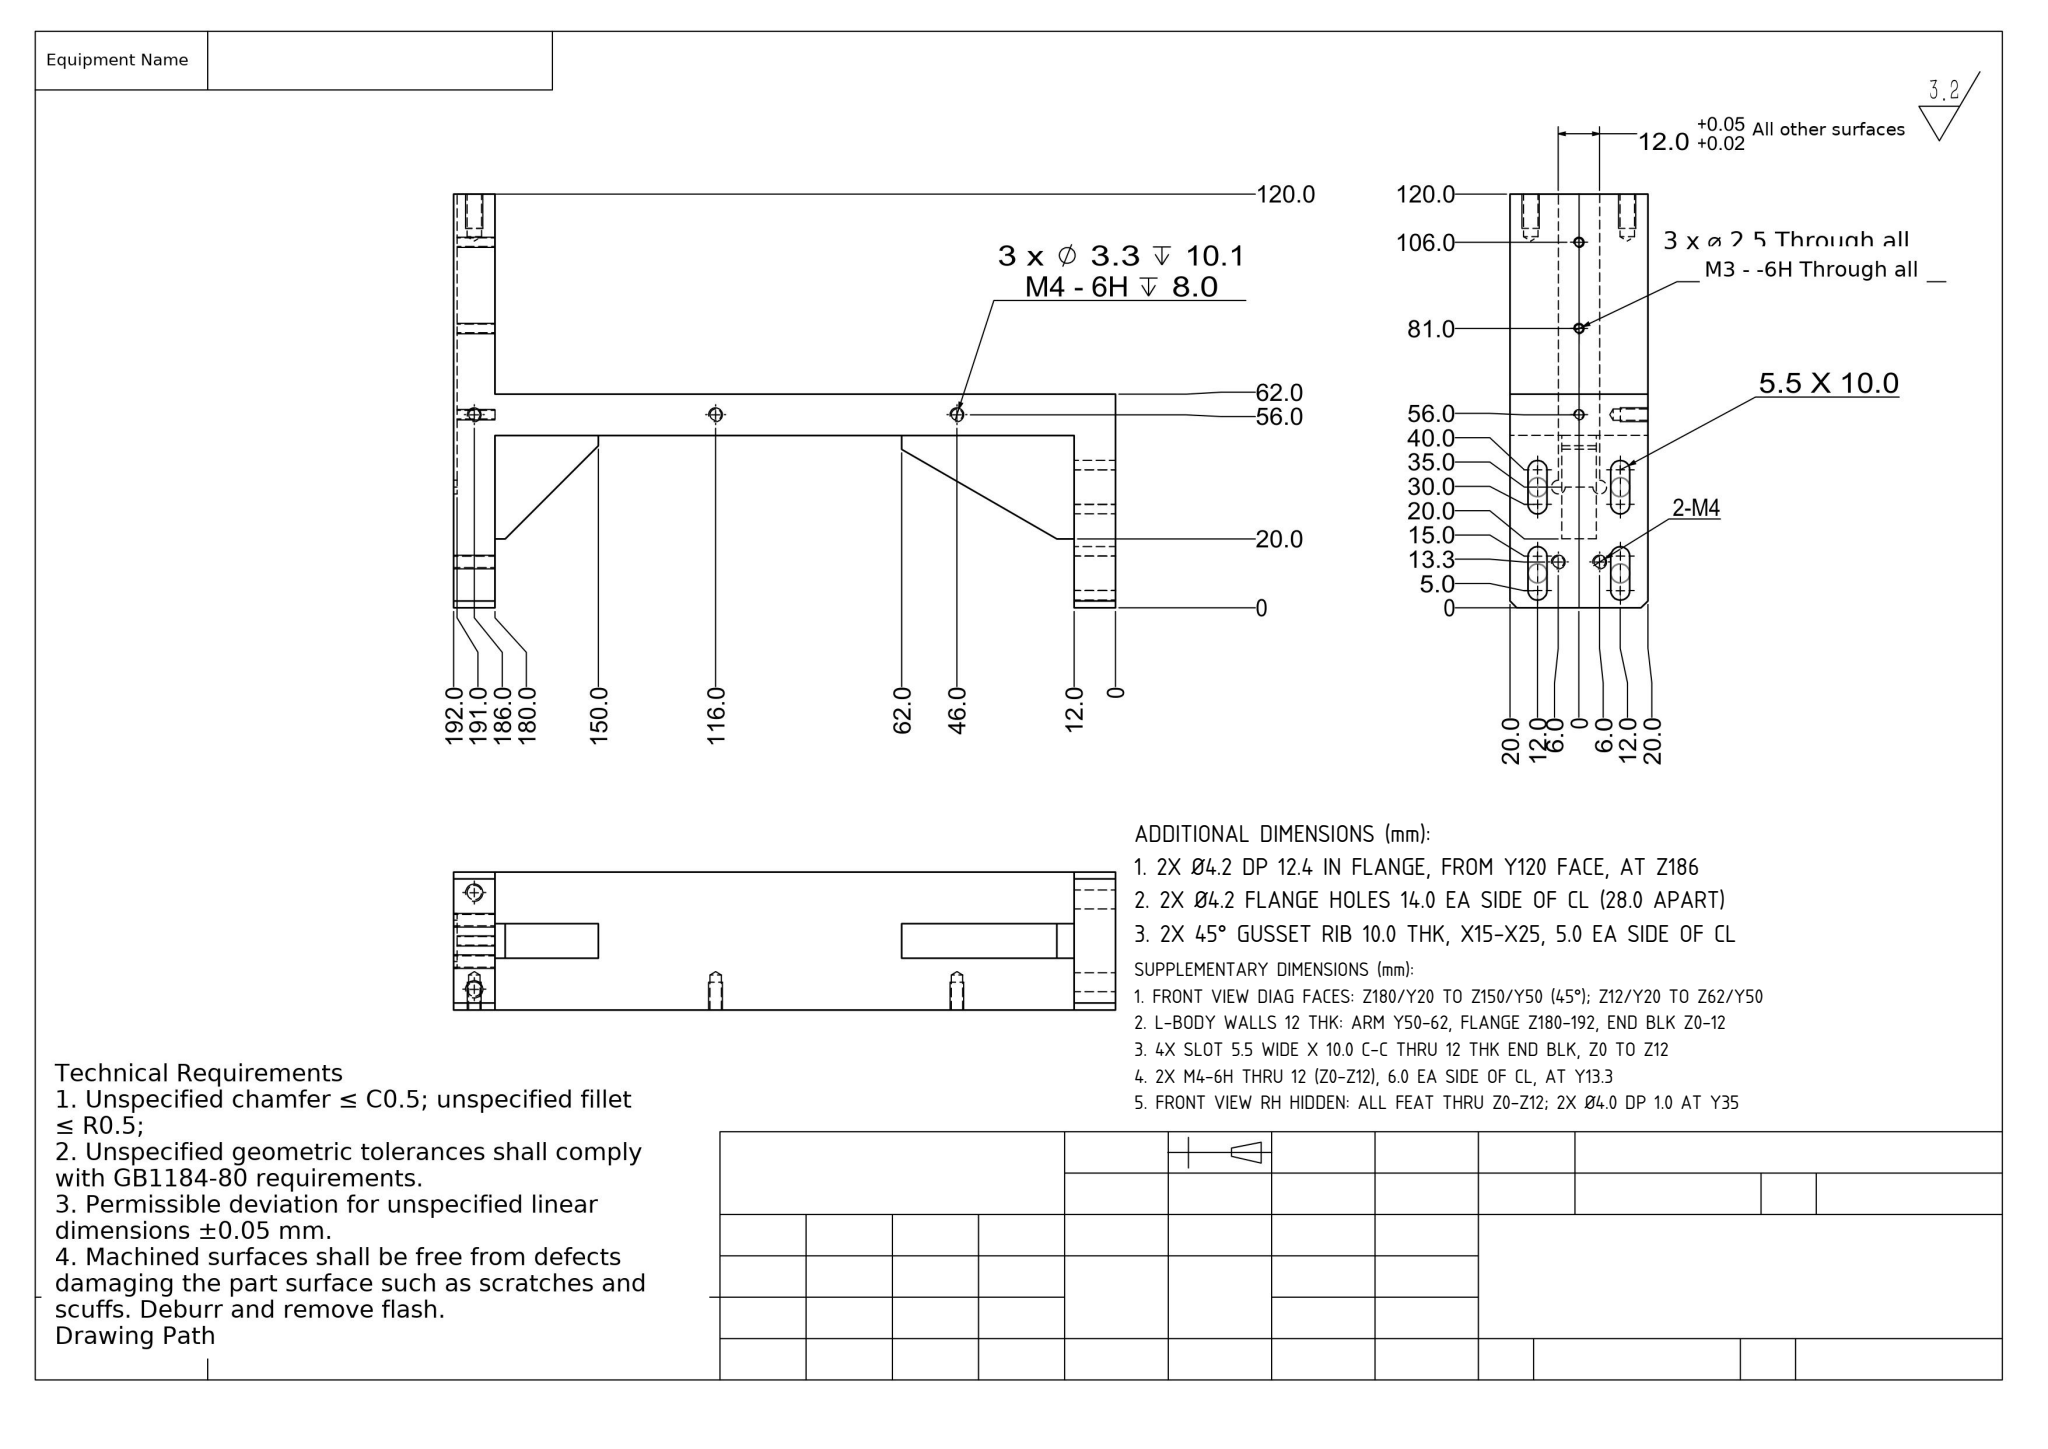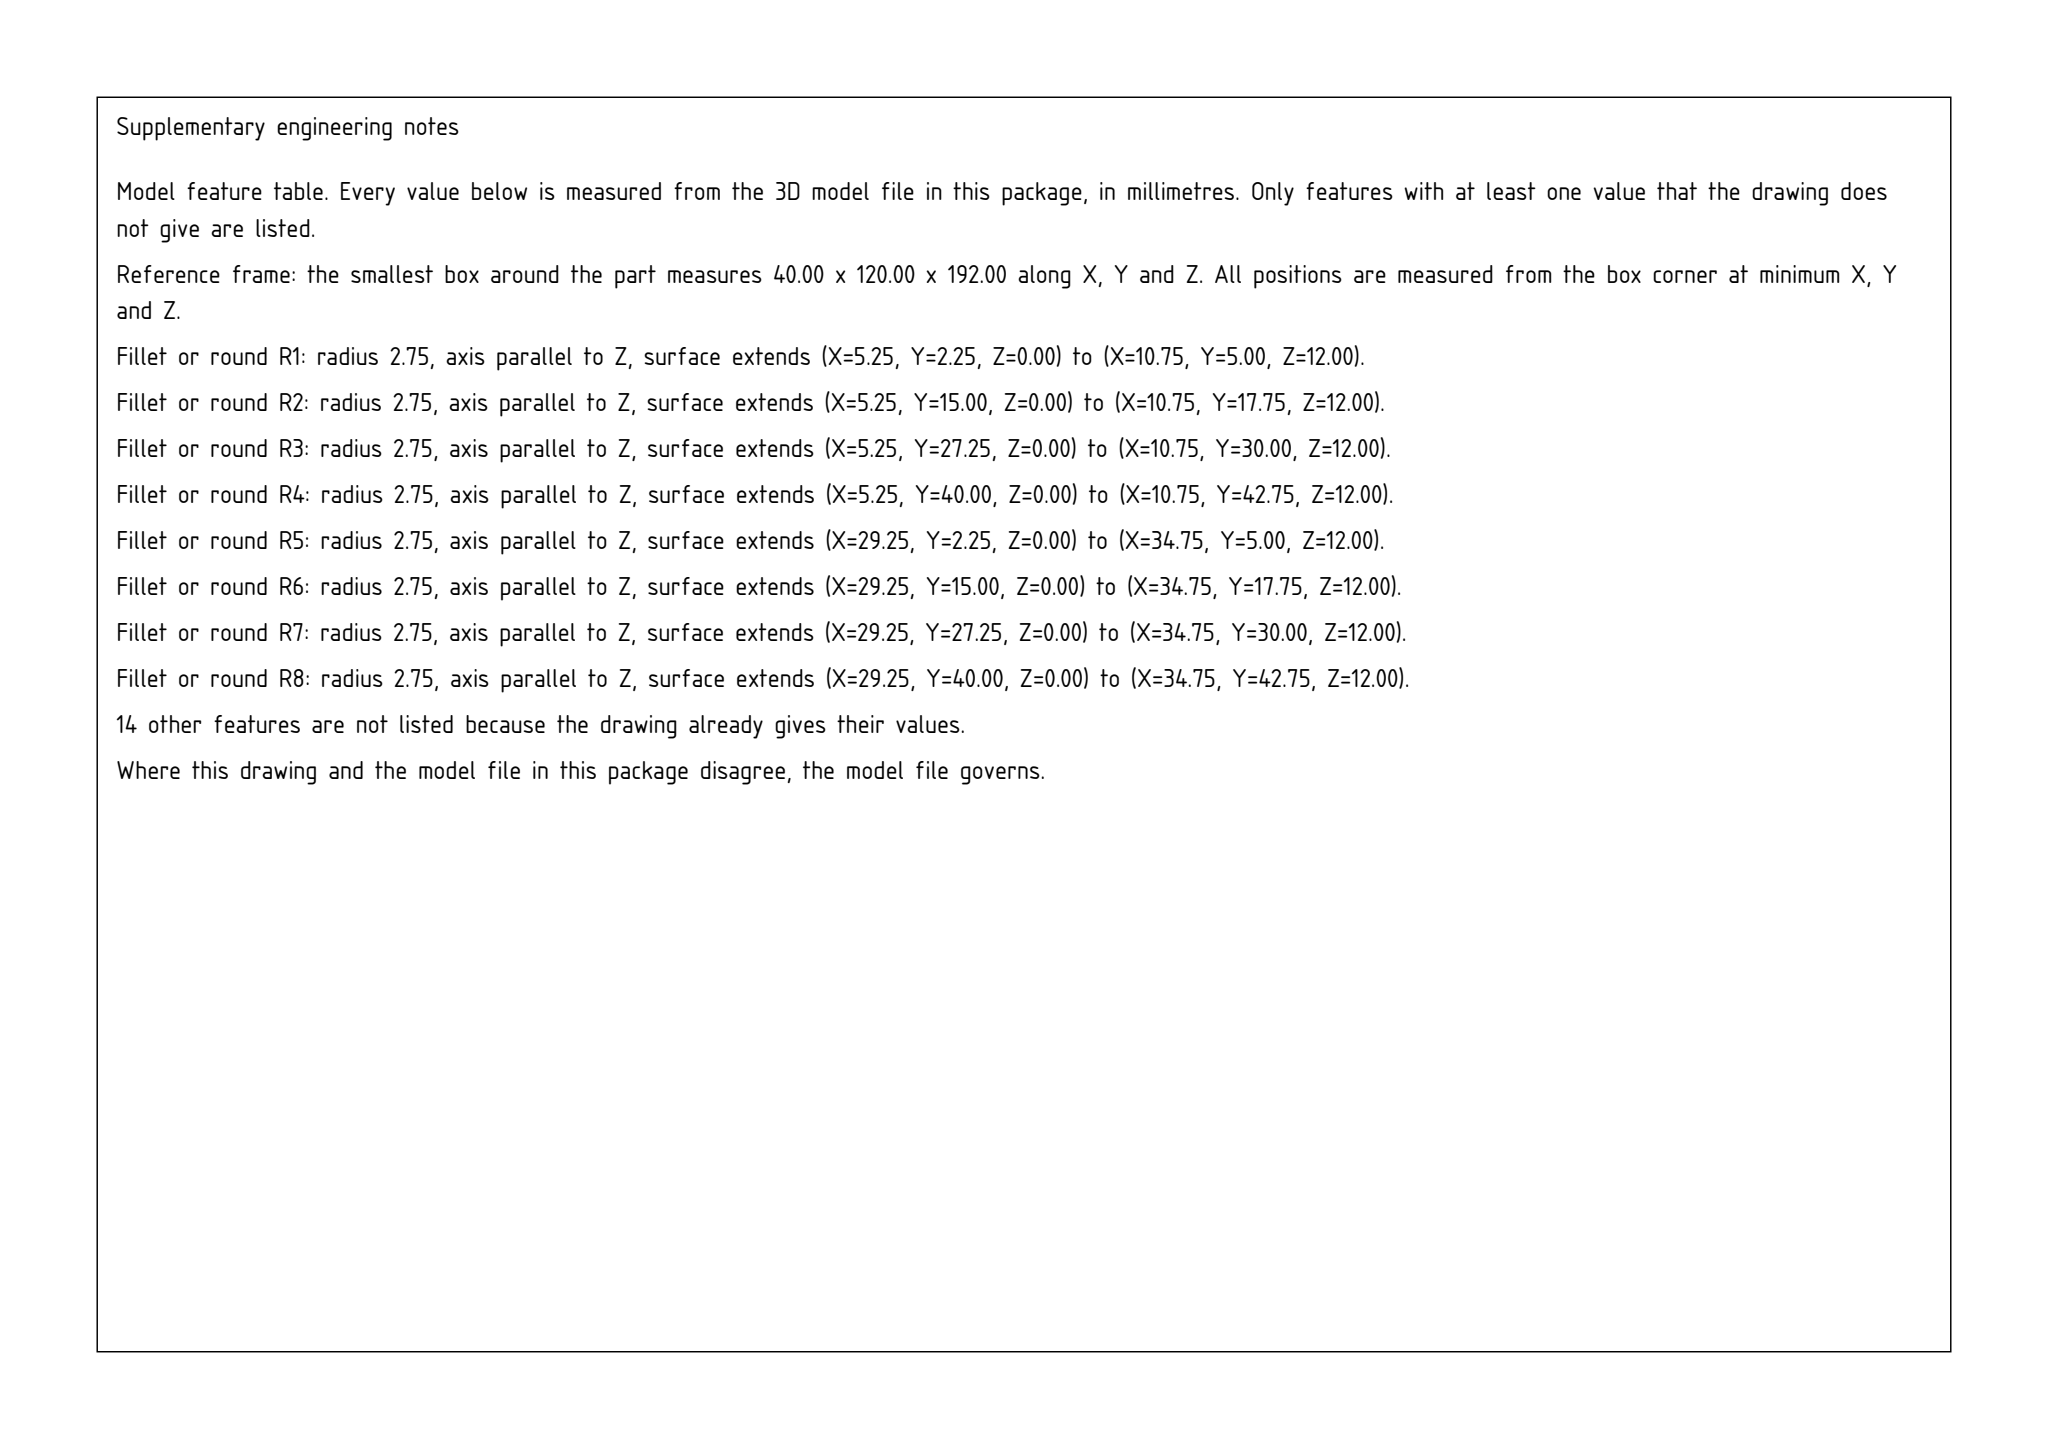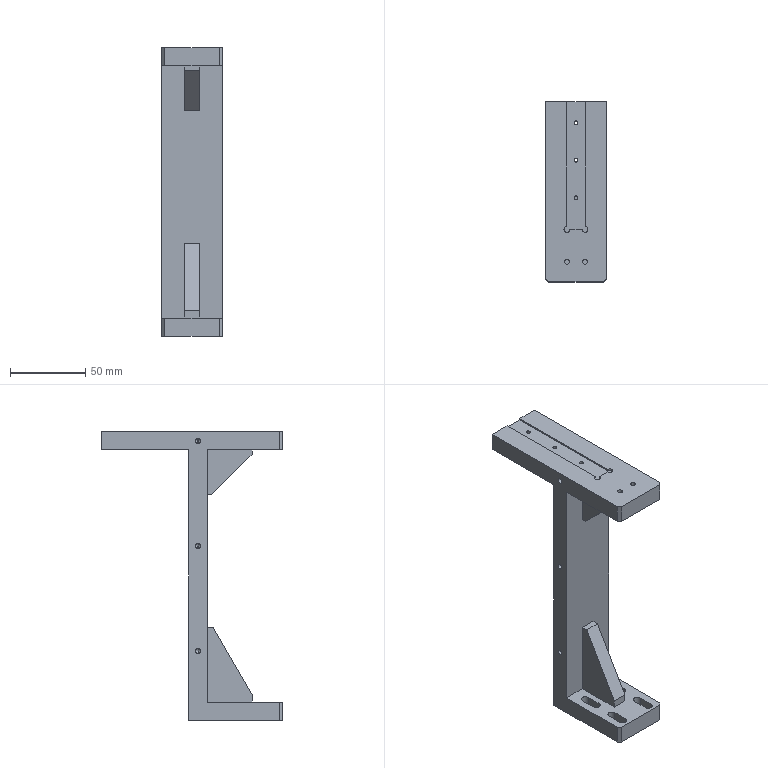Part | SolidWorks | mm | 1 solid | 80 faces | box 40 x 120 x 192 mm | volume 176604 mm3 | plane 39 | cylinder 31 | cone 10 | commonest cylinder face diameters 3.3 x10 5.5 x8 2.5 x6 4.2 x4 4 x3
build123d program:
from build123d import *

# Parameters (mm, degrees)
SKETCH1_W             = 40
SKETCH1_H             = 120
BOSS_EXTRUDE1_DEPTH   = 12
SKETCH2_W             = 12
SKETCH2_H             = 85
CUT_EXTRUDE1_DEPTH    = 1
SKETCH3_R             = 2
CUT_EXTRUDE2_DEPTH    = 10
M3_TAPPED_HOLE1_D     = 2.5
M4_TAPPED_HOLE1_D     = 3.3
SKETCH11_W            = 180
SKETCH11_H            = 12
BOSS_EXTRUDE2_DEPTH   = 40
SKETCH14_W            = 10
SKETCH14_H            = 30
BOSS_EXTRUDE3_DEPTH   = 30
CUT_EXTRUDE5_DEPTH    = 30
M4_TAPPED_HOLE3_D     = 3.3
M4_TAPPED_HOLE3_DEPTH = 10.1
M4_TAPPED_HOLE3_TIP   = 0.9914
M5_TAPPED_HOLE1_D     = 4.2
M5_TAPPED_HOLE1_DEPTH = 12.4
M5_TAPPED_HOLE1_TIP   = 1.262
SKETCH24_W            = 40
SKETCH24_H            = 50
BOSS_EXTRUDE4_DEPTH   = 12
BOSS_EXTRUDE5_DEPTH   = 10
CHAMFER1_SIZE         = 2
CUT_EXTRUDE6_DEPTH    = 12
CHAMFER2_SIZE         = 2


with BuildPart() as part:
    # Sketch1 → Boss-Extrude1 (new body)
    with BuildSketch(Plane.XY):
        with Locations((20, 60)):
            Rectangle(SKETCH1_W, SKETCH1_H)
    extrude(amount=BOSS_EXTRUDE1_DEPTH)

    # Sketch2 → Cut-Extrude1 (cut)
    with BuildSketch(Plane.XY.offset(12)):
        with Locations((20, 77.5)):
            Rectangle(SKETCH2_W, SKETCH2_H)
    extrude(amount=-CUT_EXTRUDE1_DEPTH, mode=Mode.SUBTRACT)

    # Sketch3 → Cut-Extrude2 (cut)
    with BuildSketch(Plane.XY.offset(11)):
        with Locations((26, 35)):
            Circle(SKETCH3_R)
        with Locations((14, 35)):
            Circle(SKETCH3_R)
    extrude(amount=CUT_EXTRUDE2_DEPTH, mode=Mode.SUBTRACT)

    # M3 Tapped Hole1 (through all)
    with Locations(Plane.XY.offset(11)):
        with Locations((20, 106), (20, 81), (20, 56)):
            Hole(M3_TAPPED_HOLE1_D / 2)

    # M4 Tapped Hole1 (through all)
    with Locations(Plane.XY.offset(12)):
        with Locations((14, 13.3), (26, 13.3)):
            Hole(M4_TAPPED_HOLE1_D / 2)

    # Sketch11 → Boss-Extrude2 (add)
    with BuildSketch(Plane(origin=(40, 0, 0), x_dir=(0, 0, -1), z_dir=(1, 0, 0))):
        with Locations((90, 56)):
            Rectangle(SKETCH11_W, SKETCH11_H)
    extrude(amount=-BOSS_EXTRUDE2_DEPTH)

    # Sketch14 → Boss-Extrude3 (add)
    with BuildSketch(Plane(origin=(0, 0, 0), x_dir=(-1, 0, 0), z_dir=(0, 0, -1))):
        with Locations((-20, 35)):
            Rectangle(SKETCH14_W, SKETCH14_H)
    extrude(amount=BOSS_EXTRUDE3_DEPTH)

    # Sketch15 → Cut-Extrude5 (cut)
    with BuildSketch(Plane(origin=(25, 0, 0), x_dir=(0, 0, -1), z_dir=(1, 0, 0))):
        Polygon((3, 20), (30, 47), (30, 20), align=None)
    extrude(amount=-CUT_EXTRUDE5_DEPTH, mode=Mode.SUBTRACT)

    # M4 Tapped Hole3
    with Locations(Plane(origin=(0, 0, 0), x_dir=(0, 0, -1), z_dir=(-1, 0, 0))):
        with Locations((-6, -56), (134, -56), (64, -56)):
            Hole(M4_TAPPED_HOLE3_D / 2, depth=M4_TAPPED_HOLE3_DEPTH)
            with Locations((0, 0, -(M4_TAPPED_HOLE3_DEPTH + M4_TAPPED_HOLE3_TIP / 2))):  # 118° drill point
                Cone(0, M4_TAPPED_HOLE3_D / 2, M4_TAPPED_HOLE3_TIP, mode=Mode.SUBTRACT)

    # M5 Tapped Hole1
    with Locations(Plane(origin=(0, 120, 0), x_dir=(-1, 0, 0), z_dir=(0, 1, 0))):
        with Locations((-34, 6), (-6, 6)):
            Hole(M5_TAPPED_HOLE1_D / 2, depth=M5_TAPPED_HOLE1_DEPTH)
            with Locations((0, 0, -(M5_TAPPED_HOLE1_DEPTH + M5_TAPPED_HOLE1_TIP / 2))):  # 118° drill point
                Cone(0, M5_TAPPED_HOLE1_D / 2, M5_TAPPED_HOLE1_TIP, mode=Mode.SUBTRACT)

    # Sketch24 → Boss-Extrude4 (add)
    with BuildSketch(Plane(origin=(0, 0, -180), x_dir=(-1, 0, 0), z_dir=(0, 0, -1))):
        with Locations((-20, 25)):
            Rectangle(SKETCH24_W, SKETCH24_H)
    extrude(amount=-BOSS_EXTRUDE4_DEPTH)

    # Sketch25 → Boss-Extrude5 (add)
    with BuildSketch(Plane(origin=(15, 35, 0), x_dir=(0, 1, 0), z_dir=(1, 0, 0))):
        Polygon((15, -168), (-15, -168), (-15, -163), (10.981, -118), (15, -118), align=None)
    extrude(amount=BOSS_EXTRUDE5_DEPTH)

    # Chamfer1
    chamfer1_edges = [part.edges().sort_by_distance(p)[0] for p in [
        (0, 0, -174),
        (40, 0, -174),
    ]]
    chamfer(chamfer1_edges, length=CHAMFER1_SIZE)

    # Sketch27 → Cut-Extrude6 (cut)
    with BuildSketch(Plane(origin=(0, 0, -180), x_dir=(-1, 0, 0), z_dir=(0, 0, -1))):
        with BuildLine():
            Line((-10.75, 5), (-10.75, 15))
            ThreePointArc((-10.75, 15), (-8, 17.75), (-5.25, 15))
            Line((-5.25, 15), (-5.25, 5))
            ThreePointArc((-5.25, 5), (-8, 2.25), (-10.75, 5))
        make_face()
        with BuildLine():
            Line((-29.25, 15), (-29.25, 5))
            ThreePointArc((-29.25, 5), (-32, 2.25), (-34.75, 5))
            Line((-34.75, 5), (-34.75, 15))
            ThreePointArc((-34.75, 15), (-32, 17.75), (-29.25, 15))
        make_face()
        with BuildLine():
            Line((-5.25, 40), (-5.25, 30))
            ThreePointArc((-5.25, 30), (-8, 27.25), (-10.75, 30))
            Line((-10.75, 30), (-10.75, 40))
            ThreePointArc((-10.75, 40), (-8, 42.75), (-5.25, 40))
        make_face()
        with BuildLine():
            Line((-29.25, 40), (-29.25, 30))
            ThreePointArc((-29.25, 30), (-32, 27.25), (-34.75, 30))
            Line((-34.75, 30), (-34.75, 40))
            ThreePointArc((-34.75, 40), (-32, 42.75), (-29.25, 40))
        make_face()
    extrude(amount=-CUT_EXTRUDE6_DEPTH, mode=Mode.SUBTRACT)

    # Chamfer2
    chamfer2_edges = [part.edges().sort_by_distance(p)[0] for p in [
        (0, 0, 6),
        (40, 0, 6),
    ]]
    chamfer(chamfer2_edges, length=CHAMFER2_SIZE)


solid = part.part